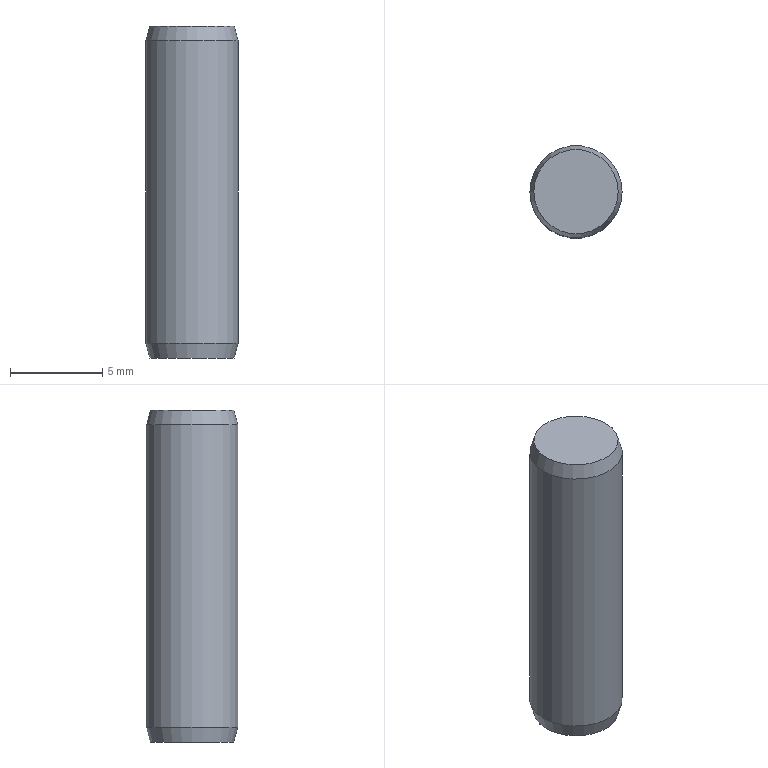Component | NX | GB-T119_1-2000_5X18_2 | 1 solid | 5 faces | box 5 x 5 x 18 mm | volume 351 mm3 | plane 2 | cone 2 | cylinder 1 | commonest cylinder face diameters 5 x1
STEP:
#1=CARTESIAN_POINT('',(0.,0.,0.));
#2=DIRECTION('',(0.,0.,1.));
#3=DIRECTION('',(1.,0.,0.));
#4=AXIS2_PLACEMENT_3D('',#1,#2,#3);
#5=CARTESIAN_POINT('',(38.214,-0.75,-25.5));
#6=VERTEX_POINT('',#5);
#7=CARTESIAN_POINT('',(40.5,-0.75,-25.5));
#8=DIRECTION('',(0.,0.,-1.));
#9=DIRECTION('',(-1.,0.,0.));
#10=AXIS2_PLACEMENT_3D('',#7,#8,#9);
#11=CIRCLE('',#10,2.286);
#12=CARTESIAN_POINT('',(40.5,-0.75,-25.5));
#13=DIRECTION('',(0.,0.,-1.));
#14=DIRECTION('',(-1.,0.,0.));
#15=AXIS2_PLACEMENT_3D('',#12,#13,#14);
#16=PLANE('',#15);
#17=CARTESIAN_POINT('',(0.,0.));
#18=DIRECTION('',(1.,0.));
#19=AXIS2_PLACEMENT_2D('',#17,#18);
#20=CIRCLE('',#19,2.286);
#21=(GEOMETRIC_REPRESENTATION_CONTEXT(2)PARAMETRIC_REPRESENTATION_CONTEXT()REPRESENTATION_CONTEXT('',''));
#22=DEFINITIONAL_REPRESENTATION('',(#20),#21);
#23=PCURVE('',#16,#22);
#24=CARTESIAN_POINT('',(40.5,-0.75,-25.5));
#25=DIRECTION('',(0.,0.,1.));
#26=DIRECTION('',(1.,0.,0.));
#27=AXIS2_PLACEMENT_3D('',#24,#25,#26);
#28=CONICAL_SURFACE('',#27,2.286,0.2618);
#29=CARTESIAN_POINT('',(9.425,-0.));
#30=DIRECTION('',(-1.,0.));
#31=VECTOR('',#30,1.);
#32=LINE('',#29,#31);
#33=(GEOMETRIC_REPRESENTATION_CONTEXT(2)PARAMETRIC_REPRESENTATION_CONTEXT()REPRESENTATION_CONTEXT('',''));
#34=DEFINITIONAL_REPRESENTATION('',(#32),#33);
#35=PCURVE('',#28,#34);
#36=SURFACE_CURVE('',#11,(#23,#35),.PCURVE_S1.);
#37=EDGE_CURVE('',#6,#6,#36,.T.);
#38=ORIENTED_EDGE('',*,*,#37,.T.);
#39=EDGE_LOOP('',(#38));
#40=FACE_BOUND('',#39,.T.);
#41=ADVANCED_FACE('',(#40),#16,.T.);
#42=CARTESIAN_POINT('',(38.,-0.75,-24.7));
#43=VERTEX_POINT('',#42);
#44=CARTESIAN_POINT('',(40.5,-0.75,-24.7));
#45=DIRECTION('',(0.,0.,-1.));
#46=DIRECTION('',(-1.,0.,0.));
#47=AXIS2_PLACEMENT_3D('',#44,#45,#46);
#48=CIRCLE('',#47,2.5);
#49=CARTESIAN_POINT('',(9.425,0.8));
#50=DIRECTION('',(-1.,0.));
#51=VECTOR('',#50,1.);
#52=LINE('',#49,#51);
#53=(GEOMETRIC_REPRESENTATION_CONTEXT(2)PARAMETRIC_REPRESENTATION_CONTEXT()REPRESENTATION_CONTEXT('',''));
#54=DEFINITIONAL_REPRESENTATION('',(#52),#53);
#55=PCURVE('',#28,#54);
#56=CARTESIAN_POINT('',(40.5,-0.75,-7.5));
#57=DIRECTION('',(0.,0.,-1.));
#58=DIRECTION('',(-1.,0.,0.));
#59=AXIS2_PLACEMENT_3D('',#56,#57,#58);
#60=CYLINDRICAL_SURFACE('',#59,2.5);
#61=CARTESIAN_POINT('',(0.,17.2));
#62=DIRECTION('',(1.,0.));
#63=VECTOR('',#62,1.);
#64=LINE('',#61,#63);
#65=(GEOMETRIC_REPRESENTATION_CONTEXT(2)PARAMETRIC_REPRESENTATION_CONTEXT()REPRESENTATION_CONTEXT('',''));
#66=DEFINITIONAL_REPRESENTATION('',(#64),#65);
#67=PCURVE('',#60,#66);
#68=SURFACE_CURVE('',#48,(#55,#67),.PCURVE_S1.);
#69=EDGE_CURVE('',#43,#43,#68,.T.);
#70=ORIENTED_EDGE('',*,*,#69,.T.);
#71=CARTESIAN_POINT('',(38.214,-0.75,-25.5));
#72=CARTESIAN_POINT('',(38.,-0.75,-24.7));
#73=B_SPLINE_CURVE_WITH_KNOTS('',1,(#71,#72),.UNSPECIFIED.,.F.,.F.,(2,2),(-0.,0.8282),.PIECEWISE_BEZIER_KNOTS.);
#74=CARTESIAN_POINT('',(3.142,0.));
#75=DIRECTION('',(0.,1.));
#76=VECTOR('',#75,1.);
#77=LINE('',#74,#76);
#78=(GEOMETRIC_REPRESENTATION_CONTEXT(2)PARAMETRIC_REPRESENTATION_CONTEXT()REPRESENTATION_CONTEXT('',''));
#79=DEFINITIONAL_REPRESENTATION('',(#77),#78);
#80=PCURVE('',#28,#79);
#81=CARTESIAN_POINT('',(9.425,0.));
#82=DIRECTION('',(0.,1.));
#83=VECTOR('',#82,1.);
#84=LINE('',#81,#83);
#85=(GEOMETRIC_REPRESENTATION_CONTEXT(2)PARAMETRIC_REPRESENTATION_CONTEXT()REPRESENTATION_CONTEXT('',''));
#86=DEFINITIONAL_REPRESENTATION('',(#84),#85);
#87=PCURVE('',#28,#86);
#88=SEAM_CURVE('',#73,(#80,#87),.PCURVE_S1.);
#89=EDGE_CURVE('',#6,#43,#88,.T.);
#90=ORIENTED_EDGE('',*,*,#89,.F.);
#91=ORIENTED_EDGE('',*,*,#37,.F.);
#92=ORIENTED_EDGE('',*,*,#89,.T.);
#93=EDGE_LOOP('',(#70,#90,#91,#92));
#94=FACE_BOUND('',#93,.T.);
#95=ADVANCED_FACE('',(#94),#28,.T.);
#96=CARTESIAN_POINT('',(38.,-0.75,-8.3));
#97=VERTEX_POINT('',#96);
#98=CARTESIAN_POINT('',(40.5,-0.75,-8.3));
#99=DIRECTION('',(0.,0.,-1.));
#100=DIRECTION('',(-1.,0.,0.));
#101=AXIS2_PLACEMENT_3D('',#98,#99,#100);
#102=CIRCLE('',#101,2.5);
#103=CARTESIAN_POINT('',(0.,0.8));
#104=DIRECTION('',(1.,0.));
#105=VECTOR('',#104,1.);
#106=LINE('',#103,#105);
#107=(GEOMETRIC_REPRESENTATION_CONTEXT(2)PARAMETRIC_REPRESENTATION_CONTEXT()REPRESENTATION_CONTEXT('',''));
#108=DEFINITIONAL_REPRESENTATION('',(#106),#107);
#109=PCURVE('',#60,#108);
#110=CARTESIAN_POINT('',(40.5,-0.75,-8.3));
#111=DIRECTION('',(0.,0.,-1.));
#112=DIRECTION('',(-1.,0.,0.));
#113=AXIS2_PLACEMENT_3D('',#110,#111,#112);
#114=CONICAL_SURFACE('',#113,2.5,0.2618);
#115=CARTESIAN_POINT('',(0.,-0.));
#116=DIRECTION('',(1.,0.));
#117=VECTOR('',#116,1.);
#118=LINE('',#115,#117);
#119=(GEOMETRIC_REPRESENTATION_CONTEXT(2)PARAMETRIC_REPRESENTATION_CONTEXT()REPRESENTATION_CONTEXT('',''));
#120=DEFINITIONAL_REPRESENTATION('',(#118),#119);
#121=PCURVE('',#114,#120);
#122=SURFACE_CURVE('',#102,(#109,#121),.PCURVE_S1.);
#123=EDGE_CURVE('',#97,#97,#122,.T.);
#124=ORIENTED_EDGE('',*,*,#123,.T.);
#125=CARTESIAN_POINT('',(38.,-0.75,-8.3));
#126=CARTESIAN_POINT('',(38.,-0.75,-24.7));
#127=B_SPLINE_CURVE_WITH_KNOTS('',1,(#125,#126),.UNSPECIFIED.,.F.,.F.,(2,2),(0.8,17.2),.PIECEWISE_BEZIER_KNOTS.);
#128=CARTESIAN_POINT('',(6.283,0.));
#129=DIRECTION('',(0.,1.));
#130=VECTOR('',#129,1.);
#131=LINE('',#128,#130);
#132=(GEOMETRIC_REPRESENTATION_CONTEXT(2)PARAMETRIC_REPRESENTATION_CONTEXT()REPRESENTATION_CONTEXT('',''));
#133=DEFINITIONAL_REPRESENTATION('',(#131),#132);
#134=PCURVE('',#60,#133);
#135=CARTESIAN_POINT('',(0.,0.));
#136=DIRECTION('',(0.,1.));
#137=VECTOR('',#136,1.);
#138=LINE('',#135,#137);
#139=(GEOMETRIC_REPRESENTATION_CONTEXT(2)PARAMETRIC_REPRESENTATION_CONTEXT()REPRESENTATION_CONTEXT('',''));
#140=DEFINITIONAL_REPRESENTATION('',(#138),#139);
#141=PCURVE('',#60,#140);
#142=SEAM_CURVE('',#127,(#134,#141),.PCURVE_S1.);
#143=EDGE_CURVE('',#97,#43,#142,.T.);
#144=ORIENTED_EDGE('',*,*,#143,.T.);
#145=ORIENTED_EDGE('',*,*,#69,.F.);
#146=ORIENTED_EDGE('',*,*,#143,.F.);
#147=EDGE_LOOP('',(#124,#144,#145,#146));
#148=FACE_BOUND('',#147,.T.);
#149=ADVANCED_FACE('',(#148),#60,.T.);
#150=CARTESIAN_POINT('',(38.214,-0.75,-7.5));
#151=VERTEX_POINT('',#150);
#152=CARTESIAN_POINT('',(40.5,-0.75,-7.5));
#153=DIRECTION('',(0.,0.,-1.));
#154=DIRECTION('',(-1.,0.,0.));
#155=AXIS2_PLACEMENT_3D('',#152,#153,#154);
#156=CIRCLE('',#155,2.286);
#157=CARTESIAN_POINT('',(0.,-0.8));
#158=DIRECTION('',(1.,0.));
#159=VECTOR('',#158,1.);
#160=LINE('',#157,#159);
#161=(GEOMETRIC_REPRESENTATION_CONTEXT(2)PARAMETRIC_REPRESENTATION_CONTEXT()REPRESENTATION_CONTEXT('',''));
#162=DEFINITIONAL_REPRESENTATION('',(#160),#161);
#163=PCURVE('',#114,#162);
#164=CARTESIAN_POINT('',(42.786,-0.75,-7.5));
#165=DIRECTION('',(0.,0.,1.));
#166=DIRECTION('',(1.,0.,0.));
#167=AXIS2_PLACEMENT_3D('',#164,#165,#166);
#168=PLANE('',#167);
#169=CARTESIAN_POINT('',(-4.571,0.));
#170=CARTESIAN_POINT('',(-4.571,3.959));
#171=CARTESIAN_POINT('',(-1.143,1.979));
#172=CARTESIAN_POINT('',(2.286,0.));
#173=CARTESIAN_POINT('',(-1.143,-1.979));
#174=CARTESIAN_POINT('',(-4.571,-3.959));
#175=CARTESIAN_POINT('',(-4.571,0.));
#176=(BOUNDED_CURVE()B_SPLINE_CURVE(2,(#169,#170,#171,#172,#173,#174,#175),.UNSPECIFIED.,.T.,.F.)B_SPLINE_CURVE_WITH_KNOTS((1,2,2,2,2,1),(-2.094,0.,2.094,4.189,6.283,8.378),.UNSPECIFIED.)CURVE()GEOMETRIC_REPRESENTATION_ITEM()RATIONAL_B_SPLINE_CURVE((1.,0.5,1.,0.5,1.,0.5,1.))REPRESENTATION_ITEM(''));
#177=(GEOMETRIC_REPRESENTATION_CONTEXT(2)PARAMETRIC_REPRESENTATION_CONTEXT()REPRESENTATION_CONTEXT('',''));
#178=DEFINITIONAL_REPRESENTATION('',(#176),#177);
#179=PCURVE('',#168,#178);
#180=SURFACE_CURVE('',#156,(#163,#179),.PCURVE_S1.);
#181=EDGE_CURVE('',#151,#151,#180,.T.);
#182=ORIENTED_EDGE('',*,*,#181,.T.);
#183=CARTESIAN_POINT('',(38.214,-0.75,-7.5));
#184=CARTESIAN_POINT('',(38.,-0.75,-8.3));
#185=B_SPLINE_CURVE_WITH_KNOTS('',1,(#183,#184),.UNSPECIFIED.,.F.,.F.,(2,2),(-0.8282,-0.),.PIECEWISE_BEZIER_KNOTS.);
#186=CARTESIAN_POINT('',(6.283,0.));
#187=DIRECTION('',(0.,1.));
#188=VECTOR('',#187,1.);
#189=LINE('',#186,#188);
#190=(GEOMETRIC_REPRESENTATION_CONTEXT(2)PARAMETRIC_REPRESENTATION_CONTEXT()REPRESENTATION_CONTEXT('',''));
#191=DEFINITIONAL_REPRESENTATION('',(#189),#190);
#192=PCURVE('',#114,#191);
#193=CARTESIAN_POINT('',(0.,0.));
#194=DIRECTION('',(0.,1.));
#195=VECTOR('',#194,1.);
#196=LINE('',#193,#195);
#197=(GEOMETRIC_REPRESENTATION_CONTEXT(2)PARAMETRIC_REPRESENTATION_CONTEXT()REPRESENTATION_CONTEXT('',''));
#198=DEFINITIONAL_REPRESENTATION('',(#196),#197);
#199=PCURVE('',#114,#198);
#200=SEAM_CURVE('',#185,(#192,#199),.PCURVE_S1.);
#201=EDGE_CURVE('',#151,#97,#200,.T.);
#202=ORIENTED_EDGE('',*,*,#201,.T.);
#203=ORIENTED_EDGE('',*,*,#123,.F.);
#204=ORIENTED_EDGE('',*,*,#201,.F.);
#205=EDGE_LOOP('',(#182,#202,#203,#204));
#206=FACE_BOUND('',#205,.T.);
#207=ADVANCED_FACE('',(#206),#114,.T.);
#208=ORIENTED_EDGE('',*,*,#181,.F.);
#209=EDGE_LOOP('',(#208));
#210=FACE_BOUND('',#209,.T.);
#211=ADVANCED_FACE('',(#210),#168,.T.);
#212=CLOSED_SHELL('',(#41,#95,#149,#207,#211));
#213=MANIFOLD_SOLID_BREP('',#212);
#214=(LENGTH_UNIT()NAMED_UNIT(*)SI_UNIT(.MILLI.,.METRE.));
#215=UNCERTAINTY_MEASURE_WITH_UNIT(LENGTH_MEASURE(0.00001),#214,'','');
#216=(NAMED_UNIT(*)PLANE_ANGLE_UNIT()SI_UNIT($,.RADIAN.));
#217=(NAMED_UNIT(*)SI_UNIT($,.STERADIAN.)SOLID_ANGLE_UNIT());
#218=(GEOMETRIC_REPRESENTATION_CONTEXT(3)GLOBAL_UNCERTAINTY_ASSIGNED_CONTEXT((#215))GLOBAL_UNIT_ASSIGNED_CONTEXT((#214,#216,#217))REPRESENTATION_CONTEXT('',''));
#219=ADVANCED_BREP_SHAPE_REPRESENTATION('',(#4,#213),#218);